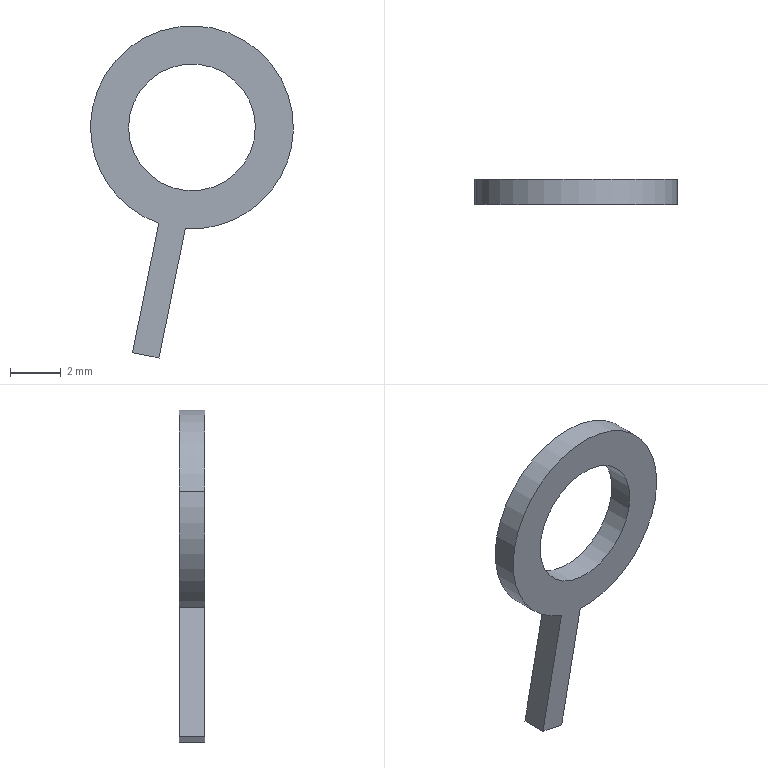Component | SolidWorks | Buckle-1 | 1 solid | 10 faces | box 8 x 1 x 13.09 mm | volume 36 mm3 | cylinder 5 | plane 5 | commonest cylinder face diameters 8 x3 5 x2
build123d program:
from build123d import *

# Parameters (mm, degrees)
BOSS_EXTRUDE2_DEPTH = 1
SKETCH2_R           = 2.5
CUT_EXTRUDE1_DEPTH  = 1


with BuildPart() as part:
    # Sketch1 → Boss-Extrude2 (new body)
    with BuildSketch(Plane(origin=(0, 0, 0), x_dir=(0, 0, -1), z_dir=(1, 0, 0))):
        with BuildLine():
            Line((-0.5352, 3.964), (-0.5352, 9.171))
            Line((-0.5352, 9.171), (0.5352, 9.171))
            Line((0.5352, 9.171), (0.5352, 3.964))
            ThreePointArc((0.5352, 3.964), (0, -4), (-0.5352, 3.964))
        make_face()
    extrude(amount=BOSS_EXTRUDE2_DEPTH)

    # Sketch2 → Cut-Extrude1 (cut)
    with BuildSketch(Plane.ZY):
        Circle(SKETCH2_R)
    extrude(amount=-CUT_EXTRUDE1_DEPTH, mode=Mode.SUBTRACT)


solid = part.part

# Placed as in the assembly
solid = solid.moved(Location((-76.689, 23.584, 193.489), (180, 78.546, 90)))
STEP:
#1=CARTESIAN_POINT('',(-2.923,0.9285,7.598));
#2=VERTEX_POINT('',#1);
#3=CARTESIAN_POINT('',(-3.116,0.9285,7.637));
#4=VERTEX_POINT('',#3);
#5=CARTESIAN_POINT('',(-3.019,0.9285,7.618));
#6=DIRECTION('',(0.,-1.,0.));
#7=DIRECTION('',(-0.9801,0.,0.1986));
#8=AXIS2_PLACEMENT_3D('',#5,#6,#7);
#9=CIRCLE('',#8,0.09843);
#10=EDGE_CURVE('',#2,#4,#9,.T.);
#11=ORIENTED_EDGE('',*,*,#10,.F.);
#12=CARTESIAN_POINT('',(-2.923,0.8891,7.598));
#13=VERTEX_POINT('',#12);
#14=CARTESIAN_POINT('',(-2.923,0.9285,7.598));
#15=DIRECTION('',(0.,-1.,0.));
#16=VECTOR('',#15,39.37);
#17=LINE('',#14,#16);
#18=EDGE_CURVE('',#2,#13,#17,.T.);
#19=ORIENTED_EDGE('',*,*,#18,.T.);
#20=CARTESIAN_POINT('',(-3.116,0.8891,7.637));
#21=VERTEX_POINT('',#20);
#22=CARTESIAN_POINT('',(-3.019,0.8891,7.618));
#23=DIRECTION('',(0.,-1.,0.));
#24=DIRECTION('',(-0.9801,0.,0.1986));
#25=AXIS2_PLACEMENT_3D('',#22,#23,#24);
#26=CIRCLE('',#25,0.09843);
#27=EDGE_CURVE('',#13,#21,#26,.T.);
#28=ORIENTED_EDGE('',*,*,#27,.T.);
#29=CARTESIAN_POINT('',(-3.116,0.9285,7.637));
#30=DIRECTION('',(0.,-1.,0.));
#31=VECTOR('',#30,39.37);
#32=LINE('',#29,#31);
#33=EDGE_CURVE('',#4,#21,#32,.T.);
#34=ORIENTED_EDGE('',*,*,#33,.F.);
#35=EDGE_LOOP('',(#11,#19,#28,#34));
#36=FACE_OUTER_BOUND('',#35,.T.);
#37=CARTESIAN_POINT('',(-3.019,0.9285,7.618));
#38=DIRECTION('',(0.,-1.,0.));
#39=DIRECTION('',(-0.9801,0.,0.1986));
#40=AXIS2_PLACEMENT_3D('',#37,#38,#39);
#41=CYLINDRICAL_SURFACE('',#40,0.09843);
#42=ADVANCED_FACE('',(#36),#41,.F.);
#43=CARTESIAN_POINT('',(-2.865,0.9285,7.586));
#44=VERTEX_POINT('',#43);
#45=CARTESIAN_POINT('',(-3.03,0.9285,7.461));
#46=VERTEX_POINT('',#45);
#47=CARTESIAN_POINT('',(-3.019,0.9285,7.618));
#48=DIRECTION('',(-0.,1.,-0.));
#49=DIRECTION('',(0.9801,0.,-0.1986));
#50=AXIS2_PLACEMENT_3D('',#47,#48,#49);
#51=CIRCLE('',#50,0.1575);
#52=EDGE_CURVE('',#44,#46,#51,.T.);
#53=ORIENTED_EDGE('',*,*,#52,.F.);
#54=CARTESIAN_POINT('',(-2.865,0.8891,7.586));
#55=VERTEX_POINT('',#54);
#56=CARTESIAN_POINT('',(-2.865,0.9285,7.586));
#57=DIRECTION('',(0.,-1.,0.));
#58=VECTOR('',#57,39.37);
#59=LINE('',#56,#58);
#60=EDGE_CURVE('',#44,#55,#59,.T.);
#61=ORIENTED_EDGE('',*,*,#60,.T.);
#62=CARTESIAN_POINT('',(-3.03,0.8891,7.461));
#63=VERTEX_POINT('',#62);
#64=CARTESIAN_POINT('',(-3.019,0.8891,7.618));
#65=DIRECTION('',(-0.,1.,-0.));
#66=DIRECTION('',(0.9801,0.,-0.1986));
#67=AXIS2_PLACEMENT_3D('',#64,#65,#66);
#68=CIRCLE('',#67,0.1575);
#69=EDGE_CURVE('',#55,#63,#68,.T.);
#70=ORIENTED_EDGE('',*,*,#69,.T.);
#71=CARTESIAN_POINT('',(-3.03,0.9285,7.461));
#72=DIRECTION('',(0.,-1.,0.));
#73=VECTOR('',#72,39.37);
#74=LINE('',#71,#73);
#75=EDGE_CURVE('',#46,#63,#74,.T.);
#76=ORIENTED_EDGE('',*,*,#75,.F.);
#77=EDGE_LOOP('',(#53,#61,#70,#76));
#78=FACE_OUTER_BOUND('',#77,.T.);
#79=CARTESIAN_POINT('',(-3.019,0.9285,7.618));
#80=DIRECTION('',(0.,-1.,0.));
#81=DIRECTION('',(-0.9801,0.,0.1986));
#82=AXIS2_PLACEMENT_3D('',#79,#80,#81);
#83=CYLINDRICAL_SURFACE('',#82,0.1575);
#84=ADVANCED_FACE('',(#78),#83,.T.);
#85=ORIENTED_EDGE('',*,*,#60,.F.);
#86=CARTESIAN_POINT('',(-3.174,0.9285,7.649));
#87=VERTEX_POINT('',#86);
#88=CARTESIAN_POINT('',(-3.019,0.9285,7.618));
#89=DIRECTION('',(-0.,1.,-0.));
#90=DIRECTION('',(0.9801,0.,-0.1986));
#91=AXIS2_PLACEMENT_3D('',#88,#89,#90);
#92=CIRCLE('',#91,0.1575);
#93=EDGE_CURVE('',#87,#44,#92,.T.);
#94=ORIENTED_EDGE('',*,*,#93,.F.);
#95=CARTESIAN_POINT('',(-3.174,0.8891,7.649));
#96=VERTEX_POINT('',#95);
#97=CARTESIAN_POINT('',(-3.174,0.9285,7.649));
#98=DIRECTION('',(0.,-1.,0.));
#99=VECTOR('',#98,39.37);
#100=LINE('',#97,#99);
#101=EDGE_CURVE('',#87,#96,#100,.T.);
#102=ORIENTED_EDGE('',*,*,#101,.T.);
#103=CARTESIAN_POINT('',(-3.019,0.8891,7.618));
#104=DIRECTION('',(-0.,1.,-0.));
#105=DIRECTION('',(0.9801,0.,-0.1986));
#106=AXIS2_PLACEMENT_3D('',#103,#104,#105);
#107=CIRCLE('',#106,0.1575);
#108=EDGE_CURVE('',#96,#55,#107,.T.);
#109=ORIENTED_EDGE('',*,*,#108,.T.);
#110=EDGE_LOOP('',(#85,#94,#102,#109));
#111=FACE_OUTER_BOUND('',#110,.T.);
#112=CARTESIAN_POINT('',(-3.019,0.9285,7.618));
#113=DIRECTION('',(0.,-1.,0.));
#114=DIRECTION('',(-0.9801,0.,0.1986));
#115=AXIS2_PLACEMENT_3D('',#112,#113,#114);
#116=CYLINDRICAL_SURFACE('',#115,0.1575);
#117=ADVANCED_FACE('',(#111),#116,.T.);
#118=CARTESIAN_POINT('',(-3.071,0.8891,7.469));
#119=VERTEX_POINT('',#118);
#120=CARTESIAN_POINT('',(-3.112,0.8891,7.268));
#121=VERTEX_POINT('',#120);
#122=CARTESIAN_POINT('',(-3.04,0.8891,7.622));
#123=DIRECTION('',(-0.1986,-0.,-0.9801));
#124=VECTOR('',#123,39.37);
#125=LINE('',#122,#124);
#126=EDGE_CURVE('',#119,#121,#125,.T.);
#127=ORIENTED_EDGE('',*,*,#126,.F.);
#128=CARTESIAN_POINT('',(-3.071,0.9285,7.469));
#129=VERTEX_POINT('',#128);
#130=CARTESIAN_POINT('',(-3.071,0.9285,7.469));
#131=DIRECTION('',(0.,-1.,0.));
#132=VECTOR('',#131,39.37);
#133=LINE('',#130,#132);
#134=EDGE_CURVE('',#129,#119,#133,.T.);
#135=ORIENTED_EDGE('',*,*,#134,.F.);
#136=CARTESIAN_POINT('',(-3.112,0.9285,7.268));
#137=VERTEX_POINT('',#136);
#138=CARTESIAN_POINT('',(-3.04,0.9285,7.622));
#139=DIRECTION('',(-0.1986,-0.,-0.9801));
#140=VECTOR('',#139,39.37);
#141=LINE('',#138,#140);
#142=EDGE_CURVE('',#129,#137,#141,.T.);
#143=ORIENTED_EDGE('',*,*,#142,.T.);
#144=CARTESIAN_POINT('',(-3.112,0.9285,7.268));
#145=DIRECTION('',(0.,-1.,0.));
#146=VECTOR('',#145,39.37);
#147=LINE('',#144,#146);
#148=EDGE_CURVE('',#137,#121,#147,.T.);
#149=ORIENTED_EDGE('',*,*,#148,.T.);
#150=EDGE_LOOP('',(#127,#135,#143,#149));
#151=FACE_OUTER_BOUND('',#150,.T.);
#152=CARTESIAN_POINT('',(-3.04,0.9285,7.622));
#153=DIRECTION('',(-0.9801,-0.,0.1986));
#154=DIRECTION('',(-0.,1.,-0.));
#155=AXIS2_PLACEMENT_3D('',#152,#153,#154);
#156=PLANE('',#155);
#157=ADVANCED_FACE('',(#151),#156,.T.);
#158=ORIENTED_EDGE('',*,*,#101,.F.);
#159=CARTESIAN_POINT('',(-3.019,0.9285,7.618));
#160=DIRECTION('',(-0.,1.,-0.));
#161=DIRECTION('',(0.9801,0.,-0.1986));
#162=AXIS2_PLACEMENT_3D('',#159,#160,#161);
#163=CIRCLE('',#162,0.1575);
#164=EDGE_CURVE('',#129,#87,#163,.T.);
#165=ORIENTED_EDGE('',*,*,#164,.F.);
#166=ORIENTED_EDGE('',*,*,#134,.T.);
#167=CARTESIAN_POINT('',(-3.019,0.8891,7.618));
#168=DIRECTION('',(-0.,1.,-0.));
#169=DIRECTION('',(0.9801,0.,-0.1986));
#170=AXIS2_PLACEMENT_3D('',#167,#168,#169);
#171=CIRCLE('',#170,0.1575);
#172=EDGE_CURVE('',#119,#96,#171,.T.);
#173=ORIENTED_EDGE('',*,*,#172,.T.);
#174=EDGE_LOOP('',(#158,#165,#166,#173));
#175=FACE_OUTER_BOUND('',#174,.T.);
#176=CARTESIAN_POINT('',(-3.019,0.9285,7.618));
#177=DIRECTION('',(0.,-1.,0.));
#178=DIRECTION('',(-0.9801,0.,0.1986));
#179=AXIS2_PLACEMENT_3D('',#176,#177,#178);
#180=CYLINDRICAL_SURFACE('',#179,0.1575);
#181=ADVANCED_FACE('',(#175),#180,.T.);
#182=CARTESIAN_POINT('',(-3.07,0.8891,7.26));
#183=VERTEX_POINT('',#182);
#184=CARTESIAN_POINT('',(-2.999,0.8891,7.613));
#185=DIRECTION('',(-0.1986,-0.,-0.9801));
#186=VECTOR('',#185,39.37);
#187=LINE('',#184,#186);
#188=EDGE_CURVE('',#63,#183,#187,.T.);
#189=ORIENTED_EDGE('',*,*,#188,.T.);
#190=CARTESIAN_POINT('',(-3.07,0.9285,7.26));
#191=VERTEX_POINT('',#190);
#192=CARTESIAN_POINT('',(-3.07,0.9285,7.26));
#193=DIRECTION('',(0.,-1.,0.));
#194=VECTOR('',#193,39.37);
#195=LINE('',#192,#194);
#196=EDGE_CURVE('',#191,#183,#195,.T.);
#197=ORIENTED_EDGE('',*,*,#196,.F.);
#198=CARTESIAN_POINT('',(-2.999,0.9285,7.613));
#199=DIRECTION('',(-0.1986,-0.,-0.9801));
#200=VECTOR('',#199,39.37);
#201=LINE('',#198,#200);
#202=EDGE_CURVE('',#46,#191,#201,.T.);
#203=ORIENTED_EDGE('',*,*,#202,.F.);
#204=ORIENTED_EDGE('',*,*,#75,.T.);
#205=EDGE_LOOP('',(#189,#197,#203,#204));
#206=FACE_OUTER_BOUND('',#205,.T.);
#207=CARTESIAN_POINT('',(-2.999,0.9285,7.613));
#208=DIRECTION('',(-0.9801,-0.,0.1986));
#209=DIRECTION('',(0.1986,0.,0.9801));
#210=AXIS2_PLACEMENT_3D('',#207,#208,#209);
#211=PLANE('',#210);
#212=ADVANCED_FACE('',(#206),#211,.F.);
#213=CARTESIAN_POINT('',(-3.091,0.8891,7.264));
#214=DIRECTION('',(0.9801,0.,-0.1986));
#215=VECTOR('',#214,39.37);
#216=LINE('',#213,#215);
#217=EDGE_CURVE('',#121,#183,#216,.T.);
#218=ORIENTED_EDGE('',*,*,#217,.F.);
#219=ORIENTED_EDGE('',*,*,#148,.F.);
#220=CARTESIAN_POINT('',(-3.091,0.9285,7.264));
#221=DIRECTION('',(0.9801,0.,-0.1986));
#222=VECTOR('',#221,39.37);
#223=LINE('',#220,#222);
#224=EDGE_CURVE('',#137,#191,#223,.T.);
#225=ORIENTED_EDGE('',*,*,#224,.T.);
#226=ORIENTED_EDGE('',*,*,#196,.T.);
#227=EDGE_LOOP('',(#218,#219,#225,#226));
#228=FACE_OUTER_BOUND('',#227,.T.);
#229=CARTESIAN_POINT('',(-3.091,0.9285,7.264));
#230=DIRECTION('',(-0.1986,-0.,-0.9801));
#231=DIRECTION('',(-0.9801,-0.,0.1986));
#232=AXIS2_PLACEMENT_3D('',#229,#230,#231);
#233=PLANE('',#232);
#234=ADVANCED_FACE('',(#228),#233,.T.);
#235=CARTESIAN_POINT('',(-3.019,0.9285,7.618));
#236=DIRECTION('',(0.,-1.,0.));
#237=DIRECTION('',(-0.9801,0.,0.1986));
#238=AXIS2_PLACEMENT_3D('',#235,#236,#237);
#239=CIRCLE('',#238,0.09843);
#240=EDGE_CURVE('',#4,#2,#239,.T.);
#241=ORIENTED_EDGE('',*,*,#240,.T.);
#242=ORIENTED_EDGE('',*,*,#10,.T.);
#243=EDGE_LOOP('',(#241,#242));
#244=FACE_BOUND('',#243,.T.);
#245=ORIENTED_EDGE('',*,*,#142,.F.);
#246=ORIENTED_EDGE('',*,*,#164,.T.);
#247=ORIENTED_EDGE('',*,*,#93,.T.);
#248=ORIENTED_EDGE('',*,*,#52,.T.);
#249=ORIENTED_EDGE('',*,*,#202,.T.);
#250=ORIENTED_EDGE('',*,*,#224,.F.);
#251=EDGE_LOOP('',(#245,#246,#247,#248,#249,#250));
#252=FACE_OUTER_BOUND('',#251,.T.);
#253=CARTESIAN_POINT('',(-3.019,0.9285,7.618));
#254=DIRECTION('',(-0.,1.,-0.));
#255=DIRECTION('',(0.9801,0.,-0.1986));
#256=AXIS2_PLACEMENT_3D('',#253,#254,#255);
#257=PLANE('',#256);
#258=ADVANCED_FACE('',(#244,#252),#257,.T.);
#259=CARTESIAN_POINT('',(-3.019,0.8891,7.618));
#260=DIRECTION('',(0.,-1.,0.));
#261=DIRECTION('',(-0.9801,0.,0.1986));
#262=AXIS2_PLACEMENT_3D('',#259,#260,#261);
#263=CIRCLE('',#262,0.09843);
#264=EDGE_CURVE('',#21,#13,#263,.T.);
#265=ORIENTED_EDGE('',*,*,#264,.F.);
#266=ORIENTED_EDGE('',*,*,#27,.F.);
#267=EDGE_LOOP('',(#265,#266));
#268=FACE_BOUND('',#267,.T.);
#269=ORIENTED_EDGE('',*,*,#126,.T.);
#270=ORIENTED_EDGE('',*,*,#217,.T.);
#271=ORIENTED_EDGE('',*,*,#188,.F.);
#272=ORIENTED_EDGE('',*,*,#69,.F.);
#273=ORIENTED_EDGE('',*,*,#108,.F.);
#274=ORIENTED_EDGE('',*,*,#172,.F.);
#275=EDGE_LOOP('',(#269,#270,#271,#272,#273,#274));
#276=FACE_OUTER_BOUND('',#275,.T.);
#277=CARTESIAN_POINT('',(-3.019,0.8891,7.618));
#278=DIRECTION('',(-0.,1.,-0.));
#279=DIRECTION('',(0.9801,0.,-0.1986));
#280=AXIS2_PLACEMENT_3D('',#277,#278,#279);
#281=PLANE('',#280);
#282=ADVANCED_FACE('',(#268,#276),#281,.F.);
#283=ORIENTED_EDGE('',*,*,#18,.F.);
#284=ORIENTED_EDGE('',*,*,#240,.F.);
#285=ORIENTED_EDGE('',*,*,#33,.T.);
#286=ORIENTED_EDGE('',*,*,#264,.T.);
#287=EDGE_LOOP('',(#283,#284,#285,#286));
#288=FACE_OUTER_BOUND('',#287,.T.);
#289=CARTESIAN_POINT('',(-3.019,0.9285,7.618));
#290=DIRECTION('',(0.,-1.,0.));
#291=DIRECTION('',(-0.9801,0.,0.1986));
#292=AXIS2_PLACEMENT_3D('',#289,#290,#291);
#293=CYLINDRICAL_SURFACE('',#292,0.09843);
#294=ADVANCED_FACE('',(#288),#293,.F.);
#295=CLOSED_SHELL('',(#42,#84,#117,#157,#181,#212,#234,#258,#282,#294));
#296=MANIFOLD_SOLID_BREP('',#295);
#297=CARTESIAN_POINT('',(0.,0.,0.));
#298=DIRECTION('',(0.,0.,1.));
#299=DIRECTION('',(1.,0.,0.));
#300=AXIS2_PLACEMENT_3D('',#297,#298,#299);
#301=(LENGTH_UNIT()NAMED_UNIT(*)SI_UNIT($,.METRE.));
#302=LENGTH_MEASURE_WITH_UNIT(LENGTH_MEASURE(0.0254),#301);
#303=DIMENSIONAL_EXPONENTS(1.,0.,0.,0.,0.,0.,0.);
#304=(CONVERSION_BASED_UNIT('',#302)LENGTH_UNIT()NAMED_UNIT(#303));
#305=UNCERTAINTY_MEASURE_WITH_UNIT(LENGTH_MEASURE(0.00001),#304,'','');
#306=(NAMED_UNIT(*)PLANE_ANGLE_UNIT()SI_UNIT($,.RADIAN.));
#307=(NAMED_UNIT(*)SI_UNIT($,.STERADIAN.)SOLID_ANGLE_UNIT());
#308=(GEOMETRIC_REPRESENTATION_CONTEXT(3)GLOBAL_UNCERTAINTY_ASSIGNED_CONTEXT((#305))GLOBAL_UNIT_ASSIGNED_CONTEXT((#304,#306,#307))REPRESENTATION_CONTEXT('',''));
#309=ADVANCED_BREP_SHAPE_REPRESENTATION('',(#296,#300),#308);
#310=COLOUR_RGB('',0.7922,0.8196,0.9333);
#311=FILL_AREA_STYLE_COLOUR('',#310);
#312=FILL_AREA_STYLE('',(#311));
#313=SURFACE_STYLE_FILL_AREA(#312);
#314=SURFACE_SIDE_STYLE('',(#313));
#315=SURFACE_STYLE_USAGE(.BOTH.,#314);
#316=PRESENTATION_STYLE_ASSIGNMENT((#315));
#317=STYLED_ITEM('',(#316),#296);
#318=(LENGTH_UNIT()NAMED_UNIT(*)SI_UNIT($,.METRE.));
#319=LENGTH_MEASURE_WITH_UNIT(LENGTH_MEASURE(0.0254),#318);
#320=DIMENSIONAL_EXPONENTS(1.,0.,0.,0.,0.,0.,0.);
#321=(CONVERSION_BASED_UNIT('',#319)LENGTH_UNIT()NAMED_UNIT(#320));
#322=UNCERTAINTY_MEASURE_WITH_UNIT(LENGTH_MEASURE(0.00001),#321,'','');
#323=(NAMED_UNIT(*)PLANE_ANGLE_UNIT()SI_UNIT($,.RADIAN.));
#324=(NAMED_UNIT(*)SI_UNIT($,.STERADIAN.)SOLID_ANGLE_UNIT());
#325=(GEOMETRIC_REPRESENTATION_CONTEXT(3)GLOBAL_UNCERTAINTY_ASSIGNED_CONTEXT((#322))GLOBAL_UNIT_ASSIGNED_CONTEXT((#321,#323,#324))REPRESENTATION_CONTEXT('',''));
#326=MECHANICAL_DESIGN_GEOMETRIC_PRESENTATION_REPRESENTATION('',(#317),#325);
#327=PRESENTATION_LAYER_ASSIGNMENT('','',(#317));